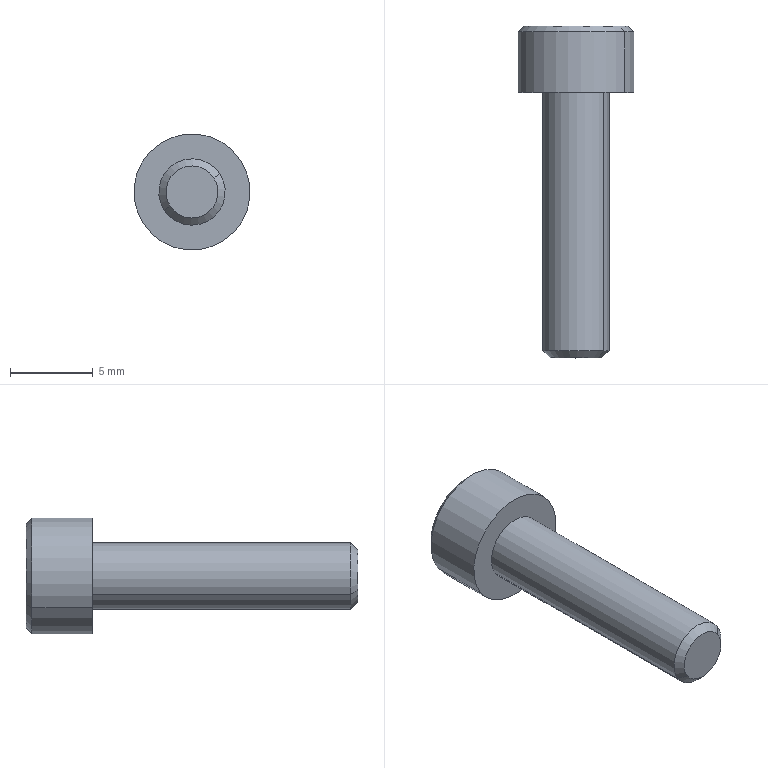Component | SolidWorks | 18M4-L16StainlessSteelScrew-1 | 1 solid | 25 faces | box 7 x 20 x 7 mm | volume 335 mm3 | plane 15 | cone 6 | cylinder 4 | commonest cylinder face diameters 4 x2 7 x2 | material SUS304
STEP:
#1=CARTESIAN_POINT('',(-0.6013,-0.04332,3.618));
#2=VERTEX_POINT('',#1);
#3=CARTESIAN_POINT('',(-0.4695,-0.04332,3.704));
#4=VERTEX_POINT('',#3);
#5=CARTESIAN_POINT('',(-0.5354,-0.04332,3.661));
#6=DIRECTION('',(0.,1.,0.));
#7=DIRECTION('',(-0.8372,0.,-0.5469));
#8=AXIS2_PLACEMENT_3D('',#5,#6,#7);
#9=CIRCLE('',#8,0.07874);
#10=EDGE_CURVE('',#2,#4,#9,.T.);
#11=ORIENTED_EDGE('',*,*,#10,.T.);
#12=CARTESIAN_POINT('',(-0.4695,0.5697,3.704));
#13=VERTEX_POINT('',#12);
#14=CARTESIAN_POINT('',(-0.4695,-0.06023,3.704));
#15=DIRECTION('',(0.,1.,0.));
#16=VECTOR('',#15,39.37);
#17=LINE('',#14,#16);
#18=EDGE_CURVE('',#4,#13,#17,.T.);
#19=ORIENTED_EDGE('',*,*,#18,.T.);
#20=CARTESIAN_POINT('',(-0.6013,0.5697,3.618));
#21=VERTEX_POINT('',#20);
#22=CARTESIAN_POINT('',(-0.5354,0.5697,3.661));
#23=DIRECTION('',(0.,-1.,0.));
#24=DIRECTION('',(-0.8372,0.,-0.5469));
#25=AXIS2_PLACEMENT_3D('',#22,#23,#24);
#26=CIRCLE('',#25,0.07874);
#27=EDGE_CURVE('',#13,#21,#26,.T.);
#28=ORIENTED_EDGE('',*,*,#27,.T.);
#29=CARTESIAN_POINT('',(-0.6013,-0.06023,3.618));
#30=DIRECTION('',(0.,1.,0.));
#31=VECTOR('',#30,39.37);
#32=LINE('',#29,#31);
#33=EDGE_CURVE('',#2,#21,#32,.T.);
#34=ORIENTED_EDGE('',*,*,#33,.F.);
#35=EDGE_LOOP('',(#11,#19,#28,#34));
#36=FACE_OUTER_BOUND('',#35,.T.);
#37=CARTESIAN_POINT('',(-0.5354,-0.06023,3.661));
#38=DIRECTION('',(0.,1.,0.));
#39=DIRECTION('',(-0.8372,0.,-0.5469));
#40=AXIS2_PLACEMENT_3D('',#37,#38,#39);
#41=CYLINDRICAL_SURFACE('',#40,0.07874);
#42=ADVANCED_FACE('',(#36),#41,.T.);
#43=CARTESIAN_POINT('',(-0.5872,-0.06023,3.628));
#44=VERTEX_POINT('',#43);
#45=CARTESIAN_POINT('',(-0.4837,-0.06023,3.695));
#46=VERTEX_POINT('',#45);
#47=CARTESIAN_POINT('',(-0.5354,-0.06023,3.661));
#48=DIRECTION('',(0.,1.,0.));
#49=DIRECTION('',(-0.8372,0.,-0.5469));
#50=AXIS2_PLACEMENT_3D('',#47,#48,#49);
#51=CIRCLE('',#50,0.06183);
#52=EDGE_CURVE('',#44,#46,#51,.T.);
#53=ORIENTED_EDGE('',*,*,#52,.T.);
#54=CARTESIAN_POINT('',(-0.4695,-0.04332,3.704));
#55=DIRECTION('',(0.592,0.7071,0.3867));
#56=VECTOR('',#55,39.37);
#57=LINE('',#54,#56);
#58=EDGE_CURVE('',#46,#4,#57,.T.);
#59=ORIENTED_EDGE('',*,*,#58,.T.);
#60=ORIENTED_EDGE('',*,*,#10,.F.);
#61=CARTESIAN_POINT('',(-0.6013,-0.04332,3.618));
#62=DIRECTION('',(-0.592,0.7071,-0.3867));
#63=VECTOR('',#62,39.37);
#64=LINE('',#61,#63);
#65=EDGE_CURVE('',#44,#2,#64,.T.);
#66=ORIENTED_EDGE('',*,*,#65,.F.);
#67=EDGE_LOOP('',(#53,#59,#60,#66));
#68=FACE_OUTER_BOUND('',#67,.T.);
#69=CARTESIAN_POINT('',(-0.5354,-0.04332,3.661));
#70=DIRECTION('',(0.,1.,0.));
#71=DIRECTION('',(-0.8372,0.,-0.5469));
#72=AXIS2_PLACEMENT_3D('',#69,#70,#71);
#73=CONICAL_SURFACE('',#72,0.07874,0.7854);
#74=ADVANCED_FACE('',(#68),#73,.T.);
#75=CARTESIAN_POINT('',(-0.6508,0.5697,3.586));
#76=VERTEX_POINT('',#75);
#77=CARTESIAN_POINT('',(-0.4201,0.5697,3.737));
#78=VERTEX_POINT('',#77);
#79=CARTESIAN_POINT('',(-0.5354,0.5697,3.661));
#80=DIRECTION('',(0.,1.,0.));
#81=DIRECTION('',(-0.8372,0.,-0.5469));
#82=AXIS2_PLACEMENT_3D('',#79,#80,#81);
#83=CIRCLE('',#82,0.1378);
#84=EDGE_CURVE('',#76,#78,#83,.T.);
#85=ORIENTED_EDGE('',*,*,#84,.T.);
#86=CARTESIAN_POINT('',(-0.4201,0.7134,3.737));
#87=VERTEX_POINT('',#86);
#88=CARTESIAN_POINT('',(-0.4201,0.5697,3.737));
#89=DIRECTION('',(0.,1.,0.));
#90=VECTOR('',#89,39.37);
#91=LINE('',#88,#90);
#92=EDGE_CURVE('',#78,#87,#91,.T.);
#93=ORIENTED_EDGE('',*,*,#92,.T.);
#94=CARTESIAN_POINT('',(-0.6508,0.7134,3.586));
#95=VERTEX_POINT('',#94);
#96=CARTESIAN_POINT('',(-0.5354,0.7134,3.661));
#97=DIRECTION('',(0.,-1.,0.));
#98=DIRECTION('',(-0.8372,0.,-0.5469));
#99=AXIS2_PLACEMENT_3D('',#96,#97,#98);
#100=CIRCLE('',#99,0.1378);
#101=EDGE_CURVE('',#87,#95,#100,.T.);
#102=ORIENTED_EDGE('',*,*,#101,.T.);
#103=CARTESIAN_POINT('',(-0.6508,0.5697,3.586));
#104=DIRECTION('',(0.,1.,0.));
#105=VECTOR('',#104,39.37);
#106=LINE('',#103,#105);
#107=EDGE_CURVE('',#76,#95,#106,.T.);
#108=ORIENTED_EDGE('',*,*,#107,.F.);
#109=EDGE_LOOP('',(#85,#93,#102,#108));
#110=FACE_OUTER_BOUND('',#109,.T.);
#111=CARTESIAN_POINT('',(-0.5354,0.5697,3.661));
#112=DIRECTION('',(0.,1.,0.));
#113=DIRECTION('',(-0.8372,0.,-0.5469));
#114=AXIS2_PLACEMENT_3D('',#111,#112,#113);
#115=CYLINDRICAL_SURFACE('',#114,0.1378);
#116=ADVANCED_FACE('',(#110),#115,.T.);
#117=CARTESIAN_POINT('',(-0.4316,0.7272,3.729));
#118=VERTEX_POINT('',#117);
#119=CARTESIAN_POINT('',(-0.6392,0.7272,3.594));
#120=VERTEX_POINT('',#119);
#121=CARTESIAN_POINT('',(-0.5354,0.7272,3.661));
#122=DIRECTION('',(0.,-1.,0.));
#123=DIRECTION('',(0.8372,0.,0.5469));
#124=AXIS2_PLACEMENT_3D('',#121,#122,#123);
#125=CIRCLE('',#124,0.124);
#126=EDGE_CURVE('',#118,#120,#125,.T.);
#127=ORIENTED_EDGE('',*,*,#126,.T.);
#128=CARTESIAN_POINT('',(-0.6508,0.7134,3.586));
#129=DIRECTION('',(-0.592,-0.7071,-0.3867));
#130=VECTOR('',#129,39.37);
#131=LINE('',#128,#130);
#132=EDGE_CURVE('',#120,#95,#131,.T.);
#133=ORIENTED_EDGE('',*,*,#132,.T.);
#134=ORIENTED_EDGE('',*,*,#101,.F.);
#135=CARTESIAN_POINT('',(-0.4201,0.7134,3.737));
#136=DIRECTION('',(0.592,-0.7071,0.3867));
#137=VECTOR('',#136,39.37);
#138=LINE('',#135,#137);
#139=EDGE_CURVE('',#118,#87,#138,.T.);
#140=ORIENTED_EDGE('',*,*,#139,.F.);
#141=EDGE_LOOP('',(#127,#133,#134,#140));
#142=FACE_OUTER_BOUND('',#141,.T.);
#143=CARTESIAN_POINT('',(-0.5354,0.7134,3.661));
#144=DIRECTION('',(0.,-1.,0.));
#145=DIRECTION('',(0.8372,0.,0.5469));
#146=AXIS2_PLACEMENT_3D('',#143,#144,#145);
#147=CONICAL_SURFACE('',#146,0.1378,0.7854);
#148=ADVANCED_FACE('',(#142),#147,.T.);
#149=CARTESIAN_POINT('',(-0.5354,0.6143,3.661));
#150=VERTEX_POINT('',#149);
#151=CARTESIAN_POINT('',(-0.5849,0.6484,3.629));
#152=VERTEX_POINT('',#151);
#153=CARTESIAN_POINT('',(-0.5849,0.6484,3.629));
#154=DIRECTION('',(-0.725,0.5,-0.4737));
#155=VECTOR('',#154,39.37);
#156=LINE('',#153,#155);
#157=EDGE_CURVE('',#150,#152,#156,.T.);
#158=ORIENTED_EDGE('',*,*,#157,.F.);
#159=CARTESIAN_POINT('',(-0.486,0.6484,3.694));
#160=VERTEX_POINT('',#159);
#161=CARTESIAN_POINT('',(-0.486,0.6484,3.694));
#162=DIRECTION('',(0.725,0.5,0.4737));
#163=VECTOR('',#162,39.37);
#164=LINE('',#161,#163);
#165=EDGE_CURVE('',#150,#160,#164,.T.);
#166=ORIENTED_EDGE('',*,*,#165,.T.);
#167=CARTESIAN_POINT('',(-0.4827,0.6484,3.635));
#168=VERTEX_POINT('',#167);
#169=CARTESIAN_POINT('',(-0.5354,0.6484,3.661));
#170=DIRECTION('',(0.,-1.,0.));
#171=DIRECTION('',(-0.8372,0.,-0.5469));
#172=AXIS2_PLACEMENT_3D('',#169,#170,#171);
#173=CIRCLE('',#172,0.05906);
#174=EDGE_CURVE('',#168,#160,#173,.T.);
#175=ORIENTED_EDGE('',*,*,#174,.F.);
#176=CARTESIAN_POINT('',(-0.5322,0.6484,3.602));
#177=VERTEX_POINT('',#176);
#178=CARTESIAN_POINT('',(-0.5354,0.6484,3.661));
#179=DIRECTION('',(0.,-1.,0.));
#180=DIRECTION('',(-0.8372,0.,-0.5469));
#181=AXIS2_PLACEMENT_3D('',#178,#179,#180);
#182=CIRCLE('',#181,0.05906);
#183=EDGE_CURVE('',#177,#168,#182,.T.);
#184=ORIENTED_EDGE('',*,*,#183,.F.);
#185=CARTESIAN_POINT('',(-0.5354,0.6484,3.661));
#186=DIRECTION('',(0.,-1.,0.));
#187=DIRECTION('',(-0.8372,0.,-0.5469));
#188=AXIS2_PLACEMENT_3D('',#185,#186,#187);
#189=CIRCLE('',#188,0.05906);
#190=EDGE_CURVE('',#152,#177,#189,.T.);
#191=ORIENTED_EDGE('',*,*,#190,.F.);
#192=EDGE_LOOP('',(#158,#166,#175,#184,#191));
#193=FACE_OUTER_BOUND('',#192,.T.);
#194=CARTESIAN_POINT('',(-0.5354,0.6484,3.661));
#195=DIRECTION('',(0.,1.,0.));
#196=DIRECTION('',(-0.8372,0.,-0.5469));
#197=AXIS2_PLACEMENT_3D('',#194,#195,#196);
#198=CONICAL_SURFACE('',#197,0.05906,1.047);
#199=ADVANCED_FACE('',(#193),#198,.F.);
#200=ORIENTED_EDGE('',*,*,#18,.F.);
#201=CARTESIAN_POINT('',(-0.5354,-0.04332,3.661));
#202=DIRECTION('',(0.,1.,0.));
#203=DIRECTION('',(-0.8372,0.,-0.5469));
#204=AXIS2_PLACEMENT_3D('',#201,#202,#203);
#205=CIRCLE('',#204,0.07874);
#206=EDGE_CURVE('',#4,#2,#205,.T.);
#207=ORIENTED_EDGE('',*,*,#206,.T.);
#208=ORIENTED_EDGE('',*,*,#33,.T.);
#209=CARTESIAN_POINT('',(-0.5354,0.5697,3.661));
#210=DIRECTION('',(0.,-1.,0.));
#211=DIRECTION('',(-0.8372,0.,-0.5469));
#212=AXIS2_PLACEMENT_3D('',#209,#210,#211);
#213=CIRCLE('',#212,0.07874);
#214=EDGE_CURVE('',#21,#13,#213,.T.);
#215=ORIENTED_EDGE('',*,*,#214,.T.);
#216=EDGE_LOOP('',(#200,#207,#208,#215));
#217=FACE_OUTER_BOUND('',#216,.T.);
#218=CARTESIAN_POINT('',(-0.5354,-0.06023,3.661));
#219=DIRECTION('',(0.,1.,0.));
#220=DIRECTION('',(-0.8372,0.,-0.5469));
#221=AXIS2_PLACEMENT_3D('',#218,#219,#220);
#222=CYLINDRICAL_SURFACE('',#221,0.07874);
#223=ADVANCED_FACE('',(#217),#222,.T.);
#224=ORIENTED_EDGE('',*,*,#84,.F.);
#225=CARTESIAN_POINT('',(-0.5354,0.5697,3.661));
#226=DIRECTION('',(0.,1.,0.));
#227=DIRECTION('',(-0.8372,0.,-0.5469));
#228=AXIS2_PLACEMENT_3D('',#225,#226,#227);
#229=CIRCLE('',#228,0.1378);
#230=EDGE_CURVE('',#78,#76,#229,.T.);
#231=ORIENTED_EDGE('',*,*,#230,.F.);
#232=EDGE_LOOP('',(#224,#231));
#233=FACE_OUTER_BOUND('',#232,.T.);
#234=ORIENTED_EDGE('',*,*,#214,.F.);
#235=ORIENTED_EDGE('',*,*,#27,.F.);
#236=EDGE_LOOP('',(#234,#235));
#237=FACE_BOUND('',#236,.T.);
#238=CARTESIAN_POINT('',(-0.6108,0.5697,3.777));
#239=DIRECTION('',(0.,1.,0.));
#240=DIRECTION('',(-0.8372,0.,-0.5469));
#241=AXIS2_PLACEMENT_3D('',#238,#239,#240);
#242=PLANE('',#241);
#243=ADVANCED_FACE('',(#233,#237),#242,.F.);
#244=ORIENTED_EDGE('',*,*,#58,.F.);
#245=CARTESIAN_POINT('',(-0.5354,-0.06023,3.661));
#246=DIRECTION('',(0.,1.,0.));
#247=DIRECTION('',(-0.8372,0.,-0.5469));
#248=AXIS2_PLACEMENT_3D('',#245,#246,#247);
#249=CIRCLE('',#248,0.06183);
#250=EDGE_CURVE('',#46,#44,#249,.T.);
#251=ORIENTED_EDGE('',*,*,#250,.T.);
#252=ORIENTED_EDGE('',*,*,#65,.T.);
#253=ORIENTED_EDGE('',*,*,#206,.F.);
#254=EDGE_LOOP('',(#244,#251,#252,#253));
#255=FACE_OUTER_BOUND('',#254,.T.);
#256=CARTESIAN_POINT('',(-0.5354,-0.04332,3.661));
#257=DIRECTION('',(0.,1.,0.));
#258=DIRECTION('',(-0.8372,0.,-0.5469));
#259=AXIS2_PLACEMENT_3D('',#256,#257,#258);
#260=CONICAL_SURFACE('',#259,0.07874,0.7854);
#261=ADVANCED_FACE('',(#255),#260,.T.);
#262=ORIENTED_EDGE('',*,*,#92,.F.);
#263=ORIENTED_EDGE('',*,*,#230,.T.);
#264=ORIENTED_EDGE('',*,*,#107,.T.);
#265=CARTESIAN_POINT('',(-0.5354,0.7134,3.661));
#266=DIRECTION('',(0.,-1.,0.));
#267=DIRECTION('',(-0.8372,0.,-0.5469));
#268=AXIS2_PLACEMENT_3D('',#265,#266,#267);
#269=CIRCLE('',#268,0.1378);
#270=EDGE_CURVE('',#95,#87,#269,.T.);
#271=ORIENTED_EDGE('',*,*,#270,.T.);
#272=EDGE_LOOP('',(#262,#263,#264,#271));
#273=FACE_OUTER_BOUND('',#272,.T.);
#274=CARTESIAN_POINT('',(-0.5354,0.5697,3.661));
#275=DIRECTION('',(0.,1.,0.));
#276=DIRECTION('',(-0.8372,0.,-0.5469));
#277=AXIS2_PLACEMENT_3D('',#274,#275,#276);
#278=CYLINDRICAL_SURFACE('',#277,0.1378);
#279=ADVANCED_FACE('',(#273),#278,.T.);
#280=ORIENTED_EDGE('',*,*,#52,.F.);
#281=ORIENTED_EDGE('',*,*,#250,.F.);
#282=EDGE_LOOP('',(#280,#281));
#283=FACE_OUTER_BOUND('',#282,.T.);
#284=CARTESIAN_POINT('',(-0.5692,-0.06023,3.713));
#285=DIRECTION('',(0.,1.,0.));
#286=DIRECTION('',(-0.8372,0.,-0.5469));
#287=AXIS2_PLACEMENT_3D('',#284,#285,#286);
#288=PLANE('',#287);
#289=ADVANCED_FACE('',(#283),#288,.F.);
#290=ORIENTED_EDGE('',*,*,#132,.F.);
#291=CARTESIAN_POINT('',(-0.5354,0.7272,3.661));
#292=DIRECTION('',(0.,-1.,0.));
#293=DIRECTION('',(0.8372,0.,0.5469));
#294=AXIS2_PLACEMENT_3D('',#291,#292,#293);
#295=CIRCLE('',#294,0.124);
#296=EDGE_CURVE('',#120,#118,#295,.T.);
#297=ORIENTED_EDGE('',*,*,#296,.T.);
#298=ORIENTED_EDGE('',*,*,#139,.T.);
#299=ORIENTED_EDGE('',*,*,#270,.F.);
#300=EDGE_LOOP('',(#290,#297,#298,#299));
#301=FACE_OUTER_BOUND('',#300,.T.);
#302=CARTESIAN_POINT('',(-0.5354,0.7134,3.661));
#303=DIRECTION('',(0.,-1.,0.));
#304=DIRECTION('',(0.8372,0.,0.5469));
#305=AXIS2_PLACEMENT_3D('',#302,#303,#304);
#306=CONICAL_SURFACE('',#305,0.1378,0.7854);
#307=ADVANCED_FACE('',(#301),#306,.T.);
#308=CARTESIAN_POINT('',(-0.4981,0.7272,3.604));
#309=VERTEX_POINT('',#308);
#310=CARTESIAN_POINT('',(-0.4673,0.7272,3.665));
#311=VERTEX_POINT('',#310);
#312=CARTESIAN_POINT('',(-0.4673,0.7272,3.665));
#313=DIRECTION('',(0.4515,0.,0.8923));
#314=VECTOR('',#313,39.37);
#315=LINE('',#312,#314);
#316=EDGE_CURVE('',#309,#311,#315,.T.);
#317=ORIENTED_EDGE('',*,*,#316,.T.);
#318=CARTESIAN_POINT('',(-0.5046,0.7272,3.722));
#319=VERTEX_POINT('',#318);
#320=CARTESIAN_POINT('',(-0.5046,0.7272,3.722));
#321=DIRECTION('',(-0.5469,0.,0.8372));
#322=VECTOR('',#321,39.37);
#323=LINE('',#320,#322);
#324=EDGE_CURVE('',#311,#319,#323,.T.);
#325=ORIENTED_EDGE('',*,*,#324,.T.);
#326=CARTESIAN_POINT('',(-0.5727,0.7272,3.719));
#327=VERTEX_POINT('',#326);
#328=CARTESIAN_POINT('',(-0.5727,0.7272,3.719));
#329=DIRECTION('',(-0.9985,0.,-0.05508));
#330=VECTOR('',#329,39.37);
#331=LINE('',#328,#330);
#332=EDGE_CURVE('',#319,#327,#331,.T.);
#333=ORIENTED_EDGE('',*,*,#332,.T.);
#334=CARTESIAN_POINT('',(-0.6035,0.7272,3.658));
#335=VERTEX_POINT('',#334);
#336=CARTESIAN_POINT('',(-0.6035,0.7272,3.658));
#337=DIRECTION('',(-0.4515,0.,-0.8923));
#338=VECTOR('',#337,39.37);
#339=LINE('',#336,#338);
#340=EDGE_CURVE('',#327,#335,#339,.T.);
#341=ORIENTED_EDGE('',*,*,#340,.T.);
#342=CARTESIAN_POINT('',(-0.5662,0.7272,3.601));
#343=VERTEX_POINT('',#342);
#344=CARTESIAN_POINT('',(-0.5662,0.7272,3.601));
#345=DIRECTION('',(0.5469,0.,-0.8372));
#346=VECTOR('',#345,39.37);
#347=LINE('',#344,#346);
#348=EDGE_CURVE('',#335,#343,#347,.T.);
#349=ORIENTED_EDGE('',*,*,#348,.T.);
#350=CARTESIAN_POINT('',(-0.4981,0.7272,3.604));
#351=DIRECTION('',(-0.9985,0.,-0.05508));
#352=VECTOR('',#351,39.37);
#353=LINE('',#350,#352);
#354=EDGE_CURVE('',#309,#343,#353,.T.);
#355=ORIENTED_EDGE('',*,*,#354,.F.);
#356=EDGE_LOOP('',(#317,#325,#333,#341,#349,#355));
#357=FACE_BOUND('',#356,.T.);
#358=ORIENTED_EDGE('',*,*,#126,.F.);
#359=ORIENTED_EDGE('',*,*,#296,.F.);
#360=EDGE_LOOP('',(#358,#359));
#361=FACE_OUTER_BOUND('',#360,.T.);
#362=CARTESIAN_POINT('',(-0.5354,0.7272,3.661));
#363=DIRECTION('',(0.,-1.,0.));
#364=DIRECTION('',(0.8372,0.,0.5469));
#365=AXIS2_PLACEMENT_3D('',#362,#363,#364);
#366=PLANE('',#365);
#367=ADVANCED_FACE('',(#357,#361),#366,.F.);
#368=CARTESIAN_POINT('',(-0.5662,0.6484,3.601));
#369=VERTEX_POINT('',#368);
#370=CARTESIAN_POINT('',(-0.5662,0.6484,3.601));
#371=DIRECTION('',(0.,1.,0.));
#372=VECTOR('',#371,39.37);
#373=LINE('',#370,#372);
#374=EDGE_CURVE('',#369,#343,#373,.T.);
#375=ORIENTED_EDGE('',*,*,#374,.F.);
#376=CARTESIAN_POINT('',(-0.4981,0.6484,3.604));
#377=DIRECTION('',(-0.9985,0.,-0.05508));
#378=VECTOR('',#377,39.37);
#379=LINE('',#376,#378);
#380=EDGE_CURVE('',#177,#369,#379,.T.);
#381=ORIENTED_EDGE('',*,*,#380,.F.);
#382=CARTESIAN_POINT('',(-0.4981,0.6484,3.604));
#383=VERTEX_POINT('',#382);
#384=CARTESIAN_POINT('',(-0.4981,0.6484,3.604));
#385=DIRECTION('',(-0.9985,0.,-0.05508));
#386=VECTOR('',#385,39.37);
#387=LINE('',#384,#386);
#388=EDGE_CURVE('',#383,#177,#387,.T.);
#389=ORIENTED_EDGE('',*,*,#388,.F.);
#390=CARTESIAN_POINT('',(-0.4981,0.6484,3.604));
#391=DIRECTION('',(0.,-1.,0.));
#392=VECTOR('',#391,39.37);
#393=LINE('',#390,#392);
#394=EDGE_CURVE('',#309,#383,#393,.T.);
#395=ORIENTED_EDGE('',*,*,#394,.F.);
#396=ORIENTED_EDGE('',*,*,#354,.T.);
#397=EDGE_LOOP('',(#375,#381,#389,#395,#396));
#398=FACE_OUTER_BOUND('',#397,.T.);
#399=CARTESIAN_POINT('',(-0.4981,0.6484,3.604));
#400=DIRECTION('',(0.05508,0.,-0.9985));
#401=DIRECTION('',(-0.9985,0.,-0.05508));
#402=AXIS2_PLACEMENT_3D('',#399,#400,#401);
#403=PLANE('',#402);
#404=ADVANCED_FACE('',(#398),#403,.F.);
#405=CARTESIAN_POINT('',(-0.6035,0.6484,3.658));
#406=VERTEX_POINT('',#405);
#407=CARTESIAN_POINT('',(-0.6035,0.6484,3.658));
#408=DIRECTION('',(0.,1.,0.));
#409=VECTOR('',#408,39.37);
#410=LINE('',#407,#409);
#411=EDGE_CURVE('',#406,#335,#410,.T.);
#412=ORIENTED_EDGE('',*,*,#411,.F.);
#413=CARTESIAN_POINT('',(-0.5662,0.6484,3.601));
#414=DIRECTION('',(-0.5469,0.,0.8372));
#415=VECTOR('',#414,39.37);
#416=LINE('',#413,#415);
#417=EDGE_CURVE('',#152,#406,#416,.T.);
#418=ORIENTED_EDGE('',*,*,#417,.F.);
#419=CARTESIAN_POINT('',(-0.5662,0.6484,3.601));
#420=DIRECTION('',(-0.5469,0.,0.8372));
#421=VECTOR('',#420,39.37);
#422=LINE('',#419,#421);
#423=EDGE_CURVE('',#369,#152,#422,.T.);
#424=ORIENTED_EDGE('',*,*,#423,.F.);
#425=ORIENTED_EDGE('',*,*,#374,.T.);
#426=ORIENTED_EDGE('',*,*,#348,.F.);
#427=EDGE_LOOP('',(#412,#418,#424,#425,#426));
#428=FACE_OUTER_BOUND('',#427,.T.);
#429=CARTESIAN_POINT('',(-0.5662,0.6484,3.601));
#430=DIRECTION('',(-0.8372,0.,-0.5469));
#431=DIRECTION('',(0.,-1.,0.));
#432=AXIS2_PLACEMENT_3D('',#429,#430,#431);
#433=PLANE('',#432);
#434=ADVANCED_FACE('',(#428),#433,.F.);
#435=ORIENTED_EDGE('',*,*,#190,.T.);
#436=ORIENTED_EDGE('',*,*,#380,.T.);
#437=ORIENTED_EDGE('',*,*,#423,.T.);
#438=EDGE_LOOP('',(#435,#436,#437));
#439=FACE_OUTER_BOUND('',#438,.T.);
#440=CARTESIAN_POINT('',(-0.5354,0.6484,3.661));
#441=DIRECTION('',(0.,1.,0.));
#442=DIRECTION('',(-0.8372,0.,-0.5469));
#443=AXIS2_PLACEMENT_3D('',#440,#441,#442);
#444=PLANE('',#443);
#445=ADVANCED_FACE('',(#439),#444,.T.);
#446=ORIENTED_EDGE('',*,*,#183,.T.);
#447=CARTESIAN_POINT('',(-0.4827,0.6484,3.635));
#448=DIRECTION('',(-0.4515,0.,-0.8923));
#449=VECTOR('',#448,39.37);
#450=LINE('',#447,#449);
#451=EDGE_CURVE('',#168,#383,#450,.T.);
#452=ORIENTED_EDGE('',*,*,#451,.T.);
#453=ORIENTED_EDGE('',*,*,#388,.T.);
#454=EDGE_LOOP('',(#446,#452,#453));
#455=FACE_OUTER_BOUND('',#454,.T.);
#456=CARTESIAN_POINT('',(-0.5354,0.6484,3.661));
#457=DIRECTION('',(0.,1.,0.));
#458=DIRECTION('',(-0.8372,0.,-0.5469));
#459=AXIS2_PLACEMENT_3D('',#456,#457,#458);
#460=PLANE('',#459);
#461=ADVANCED_FACE('',(#455),#460,.T.);
#462=ORIENTED_EDGE('',*,*,#394,.T.);
#463=ORIENTED_EDGE('',*,*,#451,.F.);
#464=CARTESIAN_POINT('',(-0.4673,0.6484,3.665));
#465=VERTEX_POINT('',#464);
#466=CARTESIAN_POINT('',(-0.4673,0.6484,3.665));
#467=DIRECTION('',(-0.4515,0.,-0.8923));
#468=VECTOR('',#467,39.37);
#469=LINE('',#466,#468);
#470=EDGE_CURVE('',#465,#168,#469,.T.);
#471=ORIENTED_EDGE('',*,*,#470,.F.);
#472=CARTESIAN_POINT('',(-0.4673,0.6484,3.665));
#473=DIRECTION('',(0.,-1.,0.));
#474=VECTOR('',#473,39.37);
#475=LINE('',#472,#474);
#476=EDGE_CURVE('',#311,#465,#475,.T.);
#477=ORIENTED_EDGE('',*,*,#476,.F.);
#478=ORIENTED_EDGE('',*,*,#316,.F.);
#479=EDGE_LOOP('',(#462,#463,#471,#477,#478));
#480=FACE_OUTER_BOUND('',#479,.T.);
#481=CARTESIAN_POINT('',(-0.4673,0.6484,3.665));
#482=DIRECTION('',(0.8923,0.,-0.4515));
#483=DIRECTION('',(-0.4515,0.,-0.8923));
#484=AXIS2_PLACEMENT_3D('',#481,#482,#483);
#485=PLANE('',#484);
#486=ADVANCED_FACE('',(#480),#485,.F.);
#487=CARTESIAN_POINT('',(-0.5727,0.6484,3.719));
#488=VERTEX_POINT('',#487);
#489=CARTESIAN_POINT('',(-0.5727,0.6484,3.719));
#490=DIRECTION('',(0.,1.,0.));
#491=VECTOR('',#490,39.37);
#492=LINE('',#489,#491);
#493=EDGE_CURVE('',#488,#327,#492,.T.);
#494=ORIENTED_EDGE('',*,*,#493,.F.);
#495=CARTESIAN_POINT('',(-0.5881,0.6484,3.688));
#496=VERTEX_POINT('',#495);
#497=CARTESIAN_POINT('',(-0.6035,0.6484,3.658));
#498=DIRECTION('',(0.4515,0.,0.8923));
#499=VECTOR('',#498,39.37);
#500=LINE('',#497,#499);
#501=EDGE_CURVE('',#496,#488,#500,.T.);
#502=ORIENTED_EDGE('',*,*,#501,.F.);
#503=CARTESIAN_POINT('',(-0.6035,0.6484,3.658));
#504=DIRECTION('',(0.4515,0.,0.8923));
#505=VECTOR('',#504,39.37);
#506=LINE('',#503,#505);
#507=EDGE_CURVE('',#406,#496,#506,.T.);
#508=ORIENTED_EDGE('',*,*,#507,.F.);
#509=ORIENTED_EDGE('',*,*,#411,.T.);
#510=ORIENTED_EDGE('',*,*,#340,.F.);
#511=EDGE_LOOP('',(#494,#502,#508,#509,#510));
#512=FACE_OUTER_BOUND('',#511,.T.);
#513=CARTESIAN_POINT('',(-0.6035,0.6484,3.658));
#514=DIRECTION('',(-0.8923,0.,0.4515));
#515=DIRECTION('',(0.4515,0.,0.8923));
#516=AXIS2_PLACEMENT_3D('',#513,#514,#515);
#517=PLANE('',#516);
#518=ADVANCED_FACE('',(#512),#517,.F.);
#519=CARTESIAN_POINT('',(-0.5354,0.6484,3.661));
#520=DIRECTION('',(0.,-1.,0.));
#521=DIRECTION('',(-0.8372,0.,-0.5469));
#522=AXIS2_PLACEMENT_3D('',#519,#520,#521);
#523=CIRCLE('',#522,0.05906);
#524=EDGE_CURVE('',#496,#152,#523,.T.);
#525=ORIENTED_EDGE('',*,*,#524,.T.);
#526=ORIENTED_EDGE('',*,*,#417,.T.);
#527=ORIENTED_EDGE('',*,*,#507,.T.);
#528=EDGE_LOOP('',(#525,#526,#527));
#529=FACE_OUTER_BOUND('',#528,.T.);
#530=CARTESIAN_POINT('',(-0.5354,0.6484,3.661));
#531=DIRECTION('',(0.,1.,0.));
#532=DIRECTION('',(-0.8372,0.,-0.5469));
#533=AXIS2_PLACEMENT_3D('',#530,#531,#532);
#534=PLANE('',#533);
#535=ADVANCED_FACE('',(#529),#534,.T.);
#536=ORIENTED_EDGE('',*,*,#165,.F.);
#537=ORIENTED_EDGE('',*,*,#157,.T.);
#538=ORIENTED_EDGE('',*,*,#524,.F.);
#539=CARTESIAN_POINT('',(-0.5387,0.6484,3.72));
#540=VERTEX_POINT('',#539);
#541=CARTESIAN_POINT('',(-0.5354,0.6484,3.661));
#542=DIRECTION('',(0.,-1.,0.));
#543=DIRECTION('',(-0.8372,0.,-0.5469));
#544=AXIS2_PLACEMENT_3D('',#541,#542,#543);
#545=CIRCLE('',#544,0.05906);
#546=EDGE_CURVE('',#540,#496,#545,.T.);
#547=ORIENTED_EDGE('',*,*,#546,.F.);
#548=CARTESIAN_POINT('',(-0.5354,0.6484,3.661));
#549=DIRECTION('',(0.,-1.,0.));
#550=DIRECTION('',(-0.8372,0.,-0.5469));
#551=AXIS2_PLACEMENT_3D('',#548,#549,#550);
#552=CIRCLE('',#551,0.05906);
#553=EDGE_CURVE('',#160,#540,#552,.T.);
#554=ORIENTED_EDGE('',*,*,#553,.F.);
#555=EDGE_LOOP('',(#536,#537,#538,#547,#554));
#556=FACE_OUTER_BOUND('',#555,.T.);
#557=CARTESIAN_POINT('',(-0.5354,0.6484,3.661));
#558=DIRECTION('',(0.,1.,0.));
#559=DIRECTION('',(-0.8372,0.,-0.5469));
#560=AXIS2_PLACEMENT_3D('',#557,#558,#559);
#561=CONICAL_SURFACE('',#560,0.05906,1.047);
#562=ADVANCED_FACE('',(#556),#561,.F.);
#563=ORIENTED_EDGE('',*,*,#174,.T.);
#564=CARTESIAN_POINT('',(-0.486,0.6484,3.694));
#565=DIRECTION('',(0.5469,0.,-0.8372));
#566=VECTOR('',#565,39.37);
#567=LINE('',#564,#566);
#568=EDGE_CURVE('',#160,#465,#567,.T.);
#569=ORIENTED_EDGE('',*,*,#568,.T.);
#570=ORIENTED_EDGE('',*,*,#470,.T.);
#571=EDGE_LOOP('',(#563,#569,#570));
#572=FACE_OUTER_BOUND('',#571,.T.);
#573=CARTESIAN_POINT('',(-0.5354,0.6484,3.661));
#574=DIRECTION('',(0.,1.,0.));
#575=DIRECTION('',(-0.8372,0.,-0.5469));
#576=AXIS2_PLACEMENT_3D('',#573,#574,#575);
#577=PLANE('',#576);
#578=ADVANCED_FACE('',(#572),#577,.T.);
#579=ORIENTED_EDGE('',*,*,#476,.T.);
#580=ORIENTED_EDGE('',*,*,#568,.F.);
#581=CARTESIAN_POINT('',(-0.5046,0.6484,3.722));
#582=VERTEX_POINT('',#581);
#583=CARTESIAN_POINT('',(-0.5046,0.6484,3.722));
#584=DIRECTION('',(0.5469,0.,-0.8372));
#585=VECTOR('',#584,39.37);
#586=LINE('',#583,#585);
#587=EDGE_CURVE('',#582,#160,#586,.T.);
#588=ORIENTED_EDGE('',*,*,#587,.F.);
#589=CARTESIAN_POINT('',(-0.5046,0.6484,3.722));
#590=DIRECTION('',(0.,-1.,0.));
#591=VECTOR('',#590,39.37);
#592=LINE('',#589,#591);
#593=EDGE_CURVE('',#319,#582,#592,.T.);
#594=ORIENTED_EDGE('',*,*,#593,.F.);
#595=ORIENTED_EDGE('',*,*,#324,.F.);
#596=EDGE_LOOP('',(#579,#580,#588,#594,#595));
#597=FACE_OUTER_BOUND('',#596,.T.);
#598=CARTESIAN_POINT('',(-0.5046,0.6484,3.722));
#599=DIRECTION('',(0.8372,0.,0.5469));
#600=DIRECTION('',(0.,1.,0.));
#601=AXIS2_PLACEMENT_3D('',#598,#599,#600);
#602=PLANE('',#601);
#603=ADVANCED_FACE('',(#597),#602,.F.);
#604=ORIENTED_EDGE('',*,*,#593,.T.);
#605=CARTESIAN_POINT('',(-0.5727,0.6484,3.719));
#606=DIRECTION('',(0.9985,0.,0.05508));
#607=VECTOR('',#606,39.37);
#608=LINE('',#605,#607);
#609=EDGE_CURVE('',#540,#582,#608,.T.);
#610=ORIENTED_EDGE('',*,*,#609,.F.);
#611=CARTESIAN_POINT('',(-0.5727,0.6484,3.719));
#612=DIRECTION('',(0.9985,0.,0.05508));
#613=VECTOR('',#612,39.37);
#614=LINE('',#611,#613);
#615=EDGE_CURVE('',#488,#540,#614,.T.);
#616=ORIENTED_EDGE('',*,*,#615,.F.);
#617=ORIENTED_EDGE('',*,*,#493,.T.);
#618=ORIENTED_EDGE('',*,*,#332,.F.);
#619=EDGE_LOOP('',(#604,#610,#616,#617,#618));
#620=FACE_OUTER_BOUND('',#619,.T.);
#621=CARTESIAN_POINT('',(-0.5727,0.6484,3.719));
#622=DIRECTION('',(-0.05508,0.,0.9985));
#623=DIRECTION('',(0.9985,0.,0.05508));
#624=AXIS2_PLACEMENT_3D('',#621,#622,#623);
#625=PLANE('',#624);
#626=ADVANCED_FACE('',(#620),#625,.F.);
#627=ORIENTED_EDGE('',*,*,#546,.T.);
#628=ORIENTED_EDGE('',*,*,#501,.T.);
#629=ORIENTED_EDGE('',*,*,#615,.T.);
#630=EDGE_LOOP('',(#627,#628,#629));
#631=FACE_OUTER_BOUND('',#630,.T.);
#632=CARTESIAN_POINT('',(-0.5354,0.6484,3.661));
#633=DIRECTION('',(0.,1.,0.));
#634=DIRECTION('',(-0.8372,0.,-0.5469));
#635=AXIS2_PLACEMENT_3D('',#632,#633,#634);
#636=PLANE('',#635);
#637=ADVANCED_FACE('',(#631),#636,.T.);
#638=ORIENTED_EDGE('',*,*,#553,.T.);
#639=ORIENTED_EDGE('',*,*,#609,.T.);
#640=ORIENTED_EDGE('',*,*,#587,.T.);
#641=EDGE_LOOP('',(#638,#639,#640));
#642=FACE_OUTER_BOUND('',#641,.T.);
#643=CARTESIAN_POINT('',(-0.5354,0.6484,3.661));
#644=DIRECTION('',(0.,1.,0.));
#645=DIRECTION('',(-0.8372,0.,-0.5469));
#646=AXIS2_PLACEMENT_3D('',#643,#644,#645);
#647=PLANE('',#646);
#648=ADVANCED_FACE('',(#642),#647,.T.);
#649=CLOSED_SHELL('',(#42,#74,#116,#148,#199,#223,#243,#261,#279,#289,#307,#367,#404,#434,#445,#461,#486,#518,#535,#562,#578,#603,#626,#637,#648));
#650=MANIFOLD_SOLID_BREP('',#649);
#651=CARTESIAN_POINT('',(0.,0.,0.));
#652=DIRECTION('',(0.,0.,1.));
#653=DIRECTION('',(1.,0.,0.));
#654=AXIS2_PLACEMENT_3D('',#651,#652,#653);
#655=(LENGTH_UNIT()NAMED_UNIT(*)SI_UNIT($,.METRE.));
#656=LENGTH_MEASURE_WITH_UNIT(LENGTH_MEASURE(0.0254),#655);
#657=DIMENSIONAL_EXPONENTS(1.,0.,0.,0.,0.,0.,0.);
#658=(CONVERSION_BASED_UNIT('',#656)LENGTH_UNIT()NAMED_UNIT(#657));
#659=UNCERTAINTY_MEASURE_WITH_UNIT(LENGTH_MEASURE(0.00001),#658,'','');
#660=(NAMED_UNIT(*)PLANE_ANGLE_UNIT()SI_UNIT($,.RADIAN.));
#661=(NAMED_UNIT(*)SI_UNIT($,.STERADIAN.)SOLID_ANGLE_UNIT());
#662=(GEOMETRIC_REPRESENTATION_CONTEXT(3)GLOBAL_UNCERTAINTY_ASSIGNED_CONTEXT((#659))GLOBAL_UNIT_ASSIGNED_CONTEXT((#658,#660,#661))REPRESENTATION_CONTEXT('',''));
#663=ADVANCED_BREP_SHAPE_REPRESENTATION('',(#650,#654),#662);
#664=COLOUR_RGB('',0.7922,0.8196,0.9333);
#665=FILL_AREA_STYLE_COLOUR('',#664);
#666=FILL_AREA_STYLE('',(#665));
#667=SURFACE_STYLE_FILL_AREA(#666);
#668=SURFACE_SIDE_STYLE('',(#667));
#669=SURFACE_STYLE_USAGE(.BOTH.,#668);
#670=PRESENTATION_STYLE_ASSIGNMENT((#669));
#671=STYLED_ITEM('',(#670),#650);
#672=PRESENTATION_LAYER_ASSIGNMENT('','',(#671));
#673=(LENGTH_UNIT()NAMED_UNIT(*)SI_UNIT($,.METRE.));
#674=LENGTH_MEASURE_WITH_UNIT(LENGTH_MEASURE(0.0254),#673);
#675=DIMENSIONAL_EXPONENTS(1.,0.,0.,0.,0.,0.,0.);
#676=(CONVERSION_BASED_UNIT('',#674)LENGTH_UNIT()NAMED_UNIT(#675));
#677=UNCERTAINTY_MEASURE_WITH_UNIT(LENGTH_MEASURE(0.00001),#676,'','');
#678=(NAMED_UNIT(*)PLANE_ANGLE_UNIT()SI_UNIT($,.RADIAN.));
#679=(NAMED_UNIT(*)SI_UNIT($,.STERADIAN.)SOLID_ANGLE_UNIT());
#680=(GEOMETRIC_REPRESENTATION_CONTEXT(3)GLOBAL_UNCERTAINTY_ASSIGNED_CONTEXT((#677))GLOBAL_UNIT_ASSIGNED_CONTEXT((#676,#678,#679))REPRESENTATION_CONTEXT('',''));
#681=MECHANICAL_DESIGN_GEOMETRIC_PRESENTATION_REPRESENTATION('',(#671),#680);